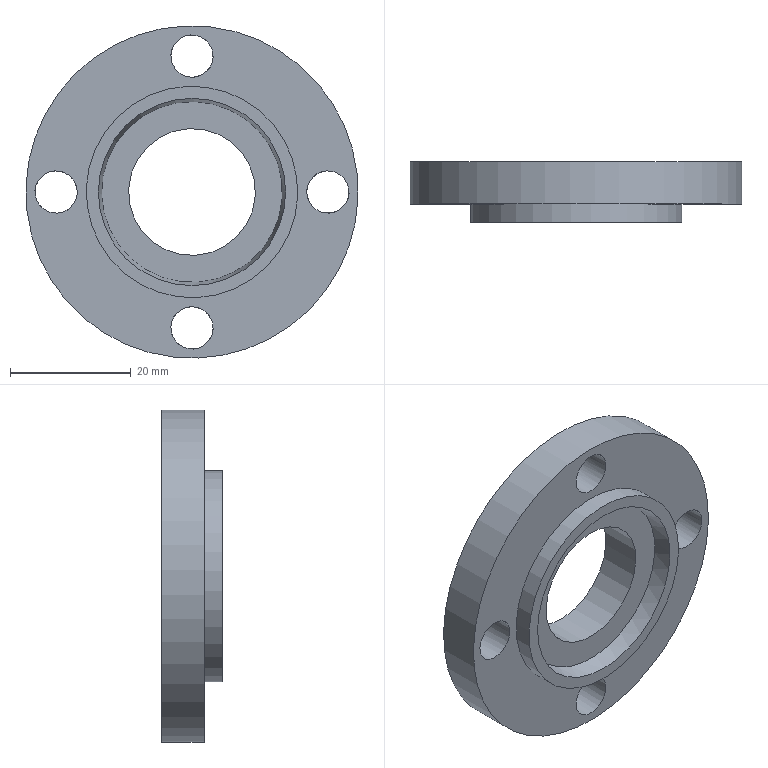Component | NX | BEARING_END_CAP_2 | 1 solid | 12 faces | box 55 x 10 x 55 mm | volume 13827 mm3 | cylinder 7 | plane 4 | cone 1 | commonest cylinder face diameters 7 x4 21 x1 35 x1 55 x1
STEP:
#1=CARTESIAN_POINT('',(0.,0.,0.));
#2=DIRECTION('',(0.,0.,1.));
#3=DIRECTION('',(1.,0.,0.));
#4=AXIS2_PLACEMENT_3D('',#1,#2,#3);
#5=CARTESIAN_POINT('',(626.689,-258.302,-1453.5));
#6=VERTEX_POINT('',#5);
#7=CARTESIAN_POINT('',(627.714,-258.302,-1451.025));
#8=VERTEX_POINT('',#7);
#9=CARTESIAN_POINT('',(630.189,-258.302,-1453.5));
#10=DIRECTION('',(0.,1.,0.));
#11=DIRECTION('',(-1.,0.,0.));
#12=AXIS2_PLACEMENT_3D('',#9,#10,#11);
#13=CIRCLE('',#12,3.5);
#14=CARTESIAN_POINT('',(610.744,-258.302,-1456.555));
#15=DIRECTION('',(0.,-1.,0.));
#16=DIRECTION('',(0.7071,0.,-0.7071));
#17=AXIS2_PLACEMENT_3D('',#14,#15,#16);
#18=PLANE('',#17);
#19=CARTESIAN_POINT('',(9.115,13.435));
#20=CARTESIAN_POINT('',(4.829,17.722));
#21=CARTESIAN_POINT('',(10.684,19.291));
#22=CARTESIAN_POINT('',(16.54,20.86));
#23=CARTESIAN_POINT('',(14.971,15.004));
#24=CARTESIAN_POINT('',(13.402,9.148));
#25=CARTESIAN_POINT('',(9.115,13.435));
#26=(BOUNDED_CURVE()B_SPLINE_CURVE(2,(#19,#20,#21,#22,#23,#24,#25),.UNSPECIFIED.,.T.,.F.)B_SPLINE_CURVE_WITH_KNOTS((1,2,2,2,2,1),(-2.094,0.,2.094,4.189,6.283,8.378),.UNSPECIFIED.)CURVE()GEOMETRIC_REPRESENTATION_ITEM()RATIONAL_B_SPLINE_CURVE((1.,0.5,1.,0.5,1.,0.5,1.))REPRESENTATION_ITEM(''));
#27=(GEOMETRIC_REPRESENTATION_CONTEXT(2)PARAMETRIC_REPRESENTATION_CONTEXT()REPRESENTATION_CONTEXT('',''));
#28=DEFINITIONAL_REPRESENTATION('',(#26),#27);
#29=PCURVE('',#18,#28);
#30=CARTESIAN_POINT('',(630.189,-281.302,-1453.5));
#31=DIRECTION('',(0.,1.,0.));
#32=DIRECTION('',(-0.7071,0.,0.7071));
#33=AXIS2_PLACEMENT_3D('',#30,#31,#32);
#34=CYLINDRICAL_SURFACE('',#33,3.5);
#35=CARTESIAN_POINT('',(5.498,23.));
#36=DIRECTION('',(1.,0.));
#37=VECTOR('',#36,1.);
#38=LINE('',#35,#37);
#39=(GEOMETRIC_REPRESENTATION_CONTEXT(2)PARAMETRIC_REPRESENTATION_CONTEXT()REPRESENTATION_CONTEXT('',''));
#40=DEFINITIONAL_REPRESENTATION('',(#38),#39);
#41=PCURVE('',#34,#40);
#42=SURFACE_CURVE('',#13,(#29,#41),.PCURVE_S1.);
#43=EDGE_CURVE('',#6,#8,#42,.T.);
#44=ORIENTED_EDGE('',*,*,#43,.F.);
#45=CARTESIAN_POINT('',(630.189,-258.302,-1453.5));
#46=DIRECTION('',(0.,1.,0.));
#47=DIRECTION('',(-1.,0.,0.));
#48=AXIS2_PLACEMENT_3D('',#45,#46,#47);
#49=CIRCLE('',#48,3.5);
#50=CARTESIAN_POINT('',(9.115,13.435));
#51=CARTESIAN_POINT('',(4.829,17.722));
#52=CARTESIAN_POINT('',(10.684,19.291));
#53=CARTESIAN_POINT('',(16.54,20.86));
#54=CARTESIAN_POINT('',(14.971,15.004));
#55=CARTESIAN_POINT('',(13.402,9.148));
#56=CARTESIAN_POINT('',(9.115,13.435));
#57=(BOUNDED_CURVE()B_SPLINE_CURVE(2,(#50,#51,#52,#53,#54,#55,#56),.UNSPECIFIED.,.T.,.F.)B_SPLINE_CURVE_WITH_KNOTS((1,2,2,2,2,1),(-2.094,0.,2.094,4.189,6.283,8.378),.UNSPECIFIED.)CURVE()GEOMETRIC_REPRESENTATION_ITEM()RATIONAL_B_SPLINE_CURVE((1.,0.5,1.,0.5,1.,0.5,1.))REPRESENTATION_ITEM(''));
#58=(GEOMETRIC_REPRESENTATION_CONTEXT(2)PARAMETRIC_REPRESENTATION_CONTEXT()REPRESENTATION_CONTEXT('',''));
#59=DEFINITIONAL_REPRESENTATION('',(#57),#58);
#60=PCURVE('',#18,#59);
#61=CARTESIAN_POINT('',(-0.7854,23.));
#62=DIRECTION('',(1.,0.));
#63=VECTOR('',#62,1.);
#64=LINE('',#61,#63);
#65=(GEOMETRIC_REPRESENTATION_CONTEXT(2)PARAMETRIC_REPRESENTATION_CONTEXT()REPRESENTATION_CONTEXT('',''));
#66=DEFINITIONAL_REPRESENTATION('',(#64),#65);
#67=PCURVE('',#34,#66);
#68=SURFACE_CURVE('',#49,(#60,#67),.PCURVE_S1.);
#69=EDGE_CURVE('',#8,#6,#68,.T.);
#70=ORIENTED_EDGE('',*,*,#69,.F.);
#71=EDGE_LOOP('',(#44,#70));
#72=FACE_BOUND('',#71,.T.);
#73=CARTESIAN_POINT('',(607.689,-258.302,-1479.5));
#74=VERTEX_POINT('',#73);
#75=CARTESIAN_POINT('',(605.214,-258.302,-1473.525));
#76=VERTEX_POINT('',#75);
#77=CARTESIAN_POINT('',(607.689,-258.302,-1476.));
#78=DIRECTION('',(0.,1.,0.));
#79=DIRECTION('',(0.,0.,-1.));
#80=AXIS2_PLACEMENT_3D('',#77,#78,#79);
#81=CIRCLE('',#80,3.5);
#82=CARTESIAN_POINT('',(14.065,-18.385));
#83=CARTESIAN_POINT('',(9.778,-22.671));
#84=CARTESIAN_POINT('',(8.209,-16.816));
#85=CARTESIAN_POINT('',(6.64,-10.96));
#86=CARTESIAN_POINT('',(12.496,-12.529));
#87=CARTESIAN_POINT('',(18.352,-14.098));
#88=CARTESIAN_POINT('',(14.065,-18.385));
#89=(BOUNDED_CURVE()B_SPLINE_CURVE(2,(#82,#83,#84,#85,#86,#87,#88),.UNSPECIFIED.,.T.,.F.)B_SPLINE_CURVE_WITH_KNOTS((1,2,2,2,2,1),(-2.094,0.,2.094,4.189,6.283,8.378),.UNSPECIFIED.)CURVE()GEOMETRIC_REPRESENTATION_ITEM()RATIONAL_B_SPLINE_CURVE((1.,0.5,1.,0.5,1.,0.5,1.))REPRESENTATION_ITEM(''));
#90=(GEOMETRIC_REPRESENTATION_CONTEXT(2)PARAMETRIC_REPRESENTATION_CONTEXT()REPRESENTATION_CONTEXT('',''));
#91=DEFINITIONAL_REPRESENTATION('',(#89),#90);
#92=PCURVE('',#18,#91);
#93=CARTESIAN_POINT('',(607.689,-281.302,-1476.));
#94=DIRECTION('',(0.,1.,0.));
#95=DIRECTION('',(-0.7071,0.,0.7071));
#96=AXIS2_PLACEMENT_3D('',#93,#94,#95);
#97=CYLINDRICAL_SURFACE('',#96,3.5);
#98=CARTESIAN_POINT('',(3.927,23.));
#99=DIRECTION('',(1.,0.));
#100=VECTOR('',#99,1.);
#101=LINE('',#98,#100);
#102=(GEOMETRIC_REPRESENTATION_CONTEXT(2)PARAMETRIC_REPRESENTATION_CONTEXT()REPRESENTATION_CONTEXT('',''));
#103=DEFINITIONAL_REPRESENTATION('',(#101),#102);
#104=PCURVE('',#97,#103);
#105=SURFACE_CURVE('',#81,(#92,#104),.PCURVE_S1.);
#106=EDGE_CURVE('',#74,#76,#105,.T.);
#107=ORIENTED_EDGE('',*,*,#106,.F.);
#108=CARTESIAN_POINT('',(607.689,-258.302,-1476.));
#109=DIRECTION('',(0.,1.,0.));
#110=DIRECTION('',(0.,0.,-1.));
#111=AXIS2_PLACEMENT_3D('',#108,#109,#110);
#112=CIRCLE('',#111,3.5);
#113=CARTESIAN_POINT('',(14.065,-18.385));
#114=CARTESIAN_POINT('',(9.778,-22.671));
#115=CARTESIAN_POINT('',(8.209,-16.816));
#116=CARTESIAN_POINT('',(6.64,-10.96));
#117=CARTESIAN_POINT('',(12.496,-12.529));
#118=CARTESIAN_POINT('',(18.352,-14.098));
#119=CARTESIAN_POINT('',(14.065,-18.385));
#120=(BOUNDED_CURVE()B_SPLINE_CURVE(2,(#113,#114,#115,#116,#117,#118,#119),.UNSPECIFIED.,.T.,.F.)B_SPLINE_CURVE_WITH_KNOTS((1,2,2,2,2,1),(-2.094,0.,2.094,4.189,6.283,8.378),.UNSPECIFIED.)CURVE()GEOMETRIC_REPRESENTATION_ITEM()RATIONAL_B_SPLINE_CURVE((1.,0.5,1.,0.5,1.,0.5,1.))REPRESENTATION_ITEM(''));
#121=(GEOMETRIC_REPRESENTATION_CONTEXT(2)PARAMETRIC_REPRESENTATION_CONTEXT()REPRESENTATION_CONTEXT('',''));
#122=DEFINITIONAL_REPRESENTATION('',(#120),#121);
#123=PCURVE('',#18,#122);
#124=CARTESIAN_POINT('',(-2.356,23.));
#125=DIRECTION('',(1.,0.));
#126=VECTOR('',#125,1.);
#127=LINE('',#124,#126);
#128=(GEOMETRIC_REPRESENTATION_CONTEXT(2)PARAMETRIC_REPRESENTATION_CONTEXT()REPRESENTATION_CONTEXT('',''));
#129=DEFINITIONAL_REPRESENTATION('',(#127),#128);
#130=PCURVE('',#97,#129);
#131=SURFACE_CURVE('',#112,(#123,#130),.PCURVE_S1.);
#132=EDGE_CURVE('',#76,#74,#131,.T.);
#133=ORIENTED_EDGE('',*,*,#132,.F.);
#134=EDGE_LOOP('',(#107,#133));
#135=FACE_BOUND('',#134,.T.);
#136=CARTESIAN_POINT('',(633.689,-258.302,-1498.5));
#137=VERTEX_POINT('',#136);
#138=CARTESIAN_POINT('',(627.714,-258.302,-1496.025));
#139=VERTEX_POINT('',#138);
#140=CARTESIAN_POINT('',(630.189,-258.302,-1498.5));
#141=DIRECTION('',(0.,1.,0.));
#142=DIRECTION('',(1.,0.,0.));
#143=AXIS2_PLACEMENT_3D('',#140,#141,#142);
#144=CIRCLE('',#143,3.5);
#145=CARTESIAN_POINT('',(45.885,-13.435));
#146=CARTESIAN_POINT('',(50.171,-17.722));
#147=CARTESIAN_POINT('',(44.316,-19.291));
#148=CARTESIAN_POINT('',(38.46,-20.86));
#149=CARTESIAN_POINT('',(40.029,-15.004));
#150=CARTESIAN_POINT('',(41.598,-9.148));
#151=CARTESIAN_POINT('',(45.885,-13.435));
#152=(BOUNDED_CURVE()B_SPLINE_CURVE(2,(#145,#146,#147,#148,#149,#150,#151),.UNSPECIFIED.,.T.,.F.)B_SPLINE_CURVE_WITH_KNOTS((1,2,2,2,2,1),(-2.094,0.,2.094,4.189,6.283,8.378),.UNSPECIFIED.)CURVE()GEOMETRIC_REPRESENTATION_ITEM()RATIONAL_B_SPLINE_CURVE((1.,0.5,1.,0.5,1.,0.5,1.))REPRESENTATION_ITEM(''));
#153=(GEOMETRIC_REPRESENTATION_CONTEXT(2)PARAMETRIC_REPRESENTATION_CONTEXT()REPRESENTATION_CONTEXT('',''));
#154=DEFINITIONAL_REPRESENTATION('',(#152),#153);
#155=PCURVE('',#18,#154);
#156=CARTESIAN_POINT('',(630.189,-281.302,-1498.5));
#157=DIRECTION('',(0.,1.,0.));
#158=DIRECTION('',(-0.7071,0.,0.7071));
#159=AXIS2_PLACEMENT_3D('',#156,#157,#158);
#160=CYLINDRICAL_SURFACE('',#159,3.5);
#161=CARTESIAN_POINT('',(2.356,23.));
#162=DIRECTION('',(1.,0.));
#163=VECTOR('',#162,1.);
#164=LINE('',#161,#163);
#165=(GEOMETRIC_REPRESENTATION_CONTEXT(2)PARAMETRIC_REPRESENTATION_CONTEXT()REPRESENTATION_CONTEXT('',''));
#166=DEFINITIONAL_REPRESENTATION('',(#164),#165);
#167=PCURVE('',#160,#166);
#168=SURFACE_CURVE('',#144,(#155,#167),.PCURVE_S1.);
#169=EDGE_CURVE('',#137,#139,#168,.T.);
#170=ORIENTED_EDGE('',*,*,#169,.F.);
#171=CARTESIAN_POINT('',(630.189,-258.302,-1498.5));
#172=DIRECTION('',(0.,1.,0.));
#173=DIRECTION('',(1.,0.,0.));
#174=AXIS2_PLACEMENT_3D('',#171,#172,#173);
#175=CIRCLE('',#174,3.5);
#176=CARTESIAN_POINT('',(45.885,-13.435));
#177=CARTESIAN_POINT('',(50.171,-17.722));
#178=CARTESIAN_POINT('',(44.316,-19.291));
#179=CARTESIAN_POINT('',(38.46,-20.86));
#180=CARTESIAN_POINT('',(40.029,-15.004));
#181=CARTESIAN_POINT('',(41.598,-9.148));
#182=CARTESIAN_POINT('',(45.885,-13.435));
#183=(BOUNDED_CURVE()B_SPLINE_CURVE(2,(#176,#177,#178,#179,#180,#181,#182),.UNSPECIFIED.,.T.,.F.)B_SPLINE_CURVE_WITH_KNOTS((1,2,2,2,2,1),(-2.094,0.,2.094,4.189,6.283,8.378),.UNSPECIFIED.)CURVE()GEOMETRIC_REPRESENTATION_ITEM()RATIONAL_B_SPLINE_CURVE((1.,0.5,1.,0.5,1.,0.5,1.))REPRESENTATION_ITEM(''));
#184=(GEOMETRIC_REPRESENTATION_CONTEXT(2)PARAMETRIC_REPRESENTATION_CONTEXT()REPRESENTATION_CONTEXT('',''));
#185=DEFINITIONAL_REPRESENTATION('',(#183),#184);
#186=PCURVE('',#18,#185);
#187=CARTESIAN_POINT('',(-3.927,23.));
#188=DIRECTION('',(1.,0.));
#189=VECTOR('',#188,1.);
#190=LINE('',#187,#189);
#191=(GEOMETRIC_REPRESENTATION_CONTEXT(2)PARAMETRIC_REPRESENTATION_CONTEXT()REPRESENTATION_CONTEXT('',''));
#192=DEFINITIONAL_REPRESENTATION('',(#190),#191);
#193=PCURVE('',#160,#192);
#194=SURFACE_CURVE('',#175,(#186,#193),.PCURVE_S1.);
#195=EDGE_CURVE('',#139,#137,#194,.T.);
#196=ORIENTED_EDGE('',*,*,#195,.F.);
#197=EDGE_LOOP('',(#170,#196));
#198=FACE_BOUND('',#197,.T.);
#199=CARTESIAN_POINT('',(652.689,-258.302,-1472.5));
#200=VERTEX_POINT('',#199);
#201=CARTESIAN_POINT('',(650.214,-258.302,-1473.525));
#202=VERTEX_POINT('',#201);
#203=CARTESIAN_POINT('',(652.689,-258.302,-1476.));
#204=DIRECTION('',(0.,1.,0.));
#205=DIRECTION('',(0.,0.,1.));
#206=AXIS2_PLACEMENT_3D('',#203,#204,#205);
#207=CIRCLE('',#206,3.5);
#208=CARTESIAN_POINT('',(40.935,18.385));
#209=CARTESIAN_POINT('',(45.222,22.671));
#210=CARTESIAN_POINT('',(46.791,16.816));
#211=CARTESIAN_POINT('',(48.36,10.96));
#212=CARTESIAN_POINT('',(42.504,12.529));
#213=CARTESIAN_POINT('',(36.648,14.098));
#214=CARTESIAN_POINT('',(40.935,18.385));
#215=(BOUNDED_CURVE()B_SPLINE_CURVE(2,(#208,#209,#210,#211,#212,#213,#214),.UNSPECIFIED.,.T.,.F.)B_SPLINE_CURVE_WITH_KNOTS((1,2,2,2,2,1),(-2.094,0.,2.094,4.189,6.283,8.378),.UNSPECIFIED.)CURVE()GEOMETRIC_REPRESENTATION_ITEM()RATIONAL_B_SPLINE_CURVE((1.,0.5,1.,0.5,1.,0.5,1.))REPRESENTATION_ITEM(''));
#216=(GEOMETRIC_REPRESENTATION_CONTEXT(2)PARAMETRIC_REPRESENTATION_CONTEXT()REPRESENTATION_CONTEXT('',''));
#217=DEFINITIONAL_REPRESENTATION('',(#215),#216);
#218=PCURVE('',#18,#217);
#219=CARTESIAN_POINT('',(652.689,-281.302,-1476.));
#220=DIRECTION('',(0.,1.,0.));
#221=DIRECTION('',(-0.7071,0.,0.7071));
#222=AXIS2_PLACEMENT_3D('',#219,#220,#221);
#223=CYLINDRICAL_SURFACE('',#222,3.5);
#224=CARTESIAN_POINT('',(0.7854,23.));
#225=DIRECTION('',(1.,0.));
#226=VECTOR('',#225,1.);
#227=LINE('',#224,#226);
#228=(GEOMETRIC_REPRESENTATION_CONTEXT(2)PARAMETRIC_REPRESENTATION_CONTEXT()REPRESENTATION_CONTEXT('',''));
#229=DEFINITIONAL_REPRESENTATION('',(#227),#228);
#230=PCURVE('',#223,#229);
#231=SURFACE_CURVE('',#207,(#218,#230),.PCURVE_S1.);
#232=EDGE_CURVE('',#200,#202,#231,.T.);
#233=ORIENTED_EDGE('',*,*,#232,.F.);
#234=CARTESIAN_POINT('',(652.689,-258.302,-1476.));
#235=DIRECTION('',(0.,1.,0.));
#236=DIRECTION('',(0.,0.,1.));
#237=AXIS2_PLACEMENT_3D('',#234,#235,#236);
#238=CIRCLE('',#237,3.5);
#239=CARTESIAN_POINT('',(40.935,18.385));
#240=CARTESIAN_POINT('',(45.222,22.671));
#241=CARTESIAN_POINT('',(46.791,16.816));
#242=CARTESIAN_POINT('',(48.36,10.96));
#243=CARTESIAN_POINT('',(42.504,12.529));
#244=CARTESIAN_POINT('',(36.648,14.098));
#245=CARTESIAN_POINT('',(40.935,18.385));
#246=(BOUNDED_CURVE()B_SPLINE_CURVE(2,(#239,#240,#241,#242,#243,#244,#245),.UNSPECIFIED.,.T.,.F.)B_SPLINE_CURVE_WITH_KNOTS((1,2,2,2,2,1),(-2.094,0.,2.094,4.189,6.283,8.378),.UNSPECIFIED.)CURVE()GEOMETRIC_REPRESENTATION_ITEM()RATIONAL_B_SPLINE_CURVE((1.,0.5,1.,0.5,1.,0.5,1.))REPRESENTATION_ITEM(''));
#247=(GEOMETRIC_REPRESENTATION_CONTEXT(2)PARAMETRIC_REPRESENTATION_CONTEXT()REPRESENTATION_CONTEXT('',''));
#248=DEFINITIONAL_REPRESENTATION('',(#246),#247);
#249=PCURVE('',#18,#248);
#250=CARTESIAN_POINT('',(-5.498,23.));
#251=DIRECTION('',(1.,0.));
#252=VECTOR('',#251,1.);
#253=LINE('',#250,#252);
#254=(GEOMETRIC_REPRESENTATION_CONTEXT(2)PARAMETRIC_REPRESENTATION_CONTEXT()REPRESENTATION_CONTEXT('',''));
#255=DEFINITIONAL_REPRESENTATION('',(#253),#254);
#256=PCURVE('',#223,#255);
#257=SURFACE_CURVE('',#238,(#249,#256),.PCURVE_S1.);
#258=EDGE_CURVE('',#202,#200,#257,.T.);
#259=ORIENTED_EDGE('',*,*,#258,.F.);
#260=EDGE_LOOP('',(#233,#259));
#261=FACE_BOUND('',#260,.T.);
#262=CARTESIAN_POINT('',(622.764,-258.302,-1468.575));
#263=VERTEX_POINT('',#262);
#264=CARTESIAN_POINT('',(630.189,-258.302,-1476.));
#265=DIRECTION('',(0.,1.,0.));
#266=DIRECTION('',(-0.7071,0.,0.7071));
#267=AXIS2_PLACEMENT_3D('',#264,#265,#266);
#268=CIRCLE('',#267,10.5);
#269=CARTESIAN_POINT('',(17.,0.));
#270=CARTESIAN_POINT('',(17.,18.187));
#271=CARTESIAN_POINT('',(32.75,9.093));
#272=CARTESIAN_POINT('',(48.5,0.));
#273=CARTESIAN_POINT('',(32.75,-9.093));
#274=CARTESIAN_POINT('',(17.,-18.187));
#275=CARTESIAN_POINT('',(17.,0.));
#276=(BOUNDED_CURVE()B_SPLINE_CURVE(2,(#269,#270,#271,#272,#273,#274,#275),.UNSPECIFIED.,.T.,.F.)B_SPLINE_CURVE_WITH_KNOTS((1,2,2,2,2,1),(-2.094,0.,2.094,4.189,6.283,8.378),.UNSPECIFIED.)CURVE()GEOMETRIC_REPRESENTATION_ITEM()RATIONAL_B_SPLINE_CURVE((1.,0.5,1.,0.5,1.,0.5,1.))REPRESENTATION_ITEM(''));
#277=(GEOMETRIC_REPRESENTATION_CONTEXT(2)PARAMETRIC_REPRESENTATION_CONTEXT()REPRESENTATION_CONTEXT('',''));
#278=DEFINITIONAL_REPRESENTATION('',(#276),#277);
#279=PCURVE('',#18,#278);
#280=CARTESIAN_POINT('',(630.189,-258.302,-1476.));
#281=DIRECTION('',(0.,1.,0.));
#282=DIRECTION('',(-0.7071,0.,0.7071));
#283=AXIS2_PLACEMENT_3D('',#280,#281,#282);
#284=CYLINDRICAL_SURFACE('',#283,10.5);
#285=CARTESIAN_POINT('',(0.,0.));
#286=DIRECTION('',(1.,0.));
#287=VECTOR('',#286,1.);
#288=LINE('',#285,#287);
#289=(GEOMETRIC_REPRESENTATION_CONTEXT(2)PARAMETRIC_REPRESENTATION_CONTEXT()REPRESENTATION_CONTEXT('',''));
#290=DEFINITIONAL_REPRESENTATION('',(#288),#289);
#291=PCURVE('',#284,#290);
#292=SURFACE_CURVE('',#268,(#279,#291),.PCURVE_S1.);
#293=EDGE_CURVE('',#263,#263,#292,.T.);
#294=ORIENTED_EDGE('',*,*,#293,.F.);
#295=EDGE_LOOP('',(#294));
#296=FACE_BOUND('',#295,.T.);
#297=CARTESIAN_POINT('',(610.744,-258.302,-1456.555));
#298=VERTEX_POINT('',#297);
#299=CARTESIAN_POINT('',(630.189,-258.302,-1476.));
#300=DIRECTION('',(0.,1.,0.));
#301=DIRECTION('',(-0.7071,0.,0.7071));
#302=AXIS2_PLACEMENT_3D('',#299,#300,#301);
#303=CIRCLE('',#302,27.5);
#304=CARTESIAN_POINT('',(-0.,0.));
#305=CARTESIAN_POINT('',(-0.,47.631));
#306=CARTESIAN_POINT('',(41.25,23.816));
#307=CARTESIAN_POINT('',(82.5,0.));
#308=CARTESIAN_POINT('',(41.25,-23.816));
#309=CARTESIAN_POINT('',(-0.,-47.631));
#310=CARTESIAN_POINT('',(-0.,0.));
#311=(BOUNDED_CURVE()B_SPLINE_CURVE(2,(#304,#305,#306,#307,#308,#309,#310),.UNSPECIFIED.,.T.,.F.)B_SPLINE_CURVE_WITH_KNOTS((1,2,2,2,2,1),(-2.094,0.,2.094,4.189,6.283,8.378),.UNSPECIFIED.)CURVE()GEOMETRIC_REPRESENTATION_ITEM()RATIONAL_B_SPLINE_CURVE((1.,0.5,1.,0.5,1.,0.5,1.))REPRESENTATION_ITEM(''));
#312=(GEOMETRIC_REPRESENTATION_CONTEXT(2)PARAMETRIC_REPRESENTATION_CONTEXT()REPRESENTATION_CONTEXT('',''));
#313=DEFINITIONAL_REPRESENTATION('',(#311),#312);
#314=PCURVE('',#18,#313);
#315=CARTESIAN_POINT('',(630.189,-258.302,-1476.));
#316=DIRECTION('',(0.,1.,0.));
#317=DIRECTION('',(-0.7071,0.,0.7071));
#318=AXIS2_PLACEMENT_3D('',#315,#316,#317);
#319=CYLINDRICAL_SURFACE('',#318,27.5);
#320=CARTESIAN_POINT('',(0.,0.));
#321=DIRECTION('',(1.,0.));
#322=VECTOR('',#321,1.);
#323=LINE('',#320,#322);
#324=(GEOMETRIC_REPRESENTATION_CONTEXT(2)PARAMETRIC_REPRESENTATION_CONTEXT()REPRESENTATION_CONTEXT('',''));
#325=DEFINITIONAL_REPRESENTATION('',(#323),#324);
#326=PCURVE('',#319,#325);
#327=SURFACE_CURVE('',#303,(#314,#326),.PCURVE_S1.);
#328=EDGE_CURVE('',#298,#298,#327,.T.);
#329=ORIENTED_EDGE('',*,*,#328,.T.);
#330=EDGE_LOOP('',(#329));
#331=FACE_BOUND('',#330,.T.);
#332=ADVANCED_FACE('',(#72,#135,#198,#261,#296,#331),#18,.F.);
#333=CARTESIAN_POINT('',(622.764,-265.302,-1468.575));
#334=VERTEX_POINT('',#333);
#335=CARTESIAN_POINT('',(630.189,-265.302,-1476.));
#336=DIRECTION('',(0.,1.,0.));
#337=DIRECTION('',(-0.7071,0.,0.7071));
#338=AXIS2_PLACEMENT_3D('',#335,#336,#337);
#339=CIRCLE('',#338,10.5);
#340=CARTESIAN_POINT('',(0.,-7.));
#341=DIRECTION('',(1.,0.));
#342=VECTOR('',#341,1.);
#343=LINE('',#340,#342);
#344=(GEOMETRIC_REPRESENTATION_CONTEXT(2)PARAMETRIC_REPRESENTATION_CONTEXT()REPRESENTATION_CONTEXT('',''));
#345=DEFINITIONAL_REPRESENTATION('',(#343),#344);
#346=PCURVE('',#284,#345);
#347=CARTESIAN_POINT('',(622.764,-265.302,-1468.575));
#348=DIRECTION('',(0.,1.,0.));
#349=DIRECTION('',(-0.7071,0.,0.7071));
#350=AXIS2_PLACEMENT_3D('',#347,#348,#349);
#351=PLANE('',#350);
#352=CARTESIAN_POINT('',(-10.5,-0.));
#353=DIRECTION('',(1.,-0.));
#354=AXIS2_PLACEMENT_2D('',#352,#353);
#355=CIRCLE('',#354,10.5);
#356=(GEOMETRIC_REPRESENTATION_CONTEXT(2)PARAMETRIC_REPRESENTATION_CONTEXT()REPRESENTATION_CONTEXT('',''));
#357=DEFINITIONAL_REPRESENTATION('',(#355),#356);
#358=PCURVE('',#351,#357);
#359=SURFACE_CURVE('',#339,(#346,#358),.PCURVE_S1.);
#360=EDGE_CURVE('',#334,#334,#359,.T.);
#361=ORIENTED_EDGE('',*,*,#360,.T.);
#362=CARTESIAN_POINT('',(622.764,-265.302,-1468.575));
#363=CARTESIAN_POINT('',(622.764,-258.302,-1468.575));
#364=B_SPLINE_CURVE_WITH_KNOTS('',1,(#362,#363),.UNSPECIFIED.,.F.,.F.,(2,2),(-7.,0.),.PIECEWISE_BEZIER_KNOTS.);
#365=CARTESIAN_POINT('',(6.283,0.));
#366=DIRECTION('',(0.,1.));
#367=VECTOR('',#366,1.);
#368=LINE('',#365,#367);
#369=(GEOMETRIC_REPRESENTATION_CONTEXT(2)PARAMETRIC_REPRESENTATION_CONTEXT()REPRESENTATION_CONTEXT('',''));
#370=DEFINITIONAL_REPRESENTATION('',(#368),#369);
#371=PCURVE('',#284,#370);
#372=CARTESIAN_POINT('',(0.,0.));
#373=DIRECTION('',(0.,1.));
#374=VECTOR('',#373,1.);
#375=LINE('',#372,#374);
#376=(GEOMETRIC_REPRESENTATION_CONTEXT(2)PARAMETRIC_REPRESENTATION_CONTEXT()REPRESENTATION_CONTEXT('',''));
#377=DEFINITIONAL_REPRESENTATION('',(#375),#376);
#378=PCURVE('',#284,#377);
#379=SEAM_CURVE('',#364,(#371,#378),.PCURVE_S1.);
#380=EDGE_CURVE('',#334,#263,#379,.T.);
#381=ORIENTED_EDGE('',*,*,#380,.T.);
#382=ORIENTED_EDGE('',*,*,#293,.F.);
#383=ORIENTED_EDGE('',*,*,#380,.F.);
#384=EDGE_LOOP('',(#361,#381,#382,#383));
#385=FACE_BOUND('',#384,.F.);
#386=ADVANCED_FACE('',(#385),#284,.F.);
#387=CARTESIAN_POINT('',(619.603,-265.302,-1465.414));
#388=VERTEX_POINT('',#387);
#389=CARTESIAN_POINT('',(630.189,-265.302,-1476.));
#390=DIRECTION('',(0.,1.,0.));
#391=DIRECTION('',(-0.7071,0.,0.7071));
#392=AXIS2_PLACEMENT_3D('',#389,#390,#391);
#393=CIRCLE('',#392,14.971);
#394=CARTESIAN_POINT('',(-10.5,-0.));
#395=DIRECTION('',(1.,0.));
#396=AXIS2_PLACEMENT_2D('',#394,#395);
#397=CIRCLE('',#396,14.971);
#398=(GEOMETRIC_REPRESENTATION_CONTEXT(2)PARAMETRIC_REPRESENTATION_CONTEXT()REPRESENTATION_CONTEXT('',''));
#399=DEFINITIONAL_REPRESENTATION('',(#397),#398);
#400=PCURVE('',#351,#399);
#401=CARTESIAN_POINT('',(630.189,-265.302,-1476.));
#402=DIRECTION('',(0.,-1.,0.));
#403=DIRECTION('',(0.7071,0.,-0.7071));
#404=AXIS2_PLACEMENT_3D('',#401,#402,#403);
#405=CONICAL_SURFACE('',#404,14.971,0.1745);
#406=CARTESIAN_POINT('',(9.425,-0.));
#407=DIRECTION('',(-1.,0.));
#408=VECTOR('',#407,1.);
#409=LINE('',#406,#408);
#410=(GEOMETRIC_REPRESENTATION_CONTEXT(2)PARAMETRIC_REPRESENTATION_CONTEXT()REPRESENTATION_CONTEXT('',''));
#411=DEFINITIONAL_REPRESENTATION('',(#409),#410);
#412=PCURVE('',#405,#411);
#413=SURFACE_CURVE('',#393,(#400,#412),.PCURVE_S1.);
#414=EDGE_CURVE('',#388,#388,#413,.T.);
#415=ORIENTED_EDGE('',*,*,#414,.F.);
#416=EDGE_LOOP('',(#415));
#417=FACE_BOUND('',#416,.T.);
#418=ORIENTED_EDGE('',*,*,#360,.T.);
#419=EDGE_LOOP('',(#418));
#420=FACE_BOUND('',#419,.T.);
#421=ADVANCED_FACE('',(#417,#420),#351,.F.);
#422=CARTESIAN_POINT('',(619.229,-268.302,-1465.04));
#423=VERTEX_POINT('',#422);
#424=CARTESIAN_POINT('',(630.189,-268.302,-1476.));
#425=DIRECTION('',(0.,1.,0.));
#426=DIRECTION('',(-0.7071,0.,0.7071));
#427=AXIS2_PLACEMENT_3D('',#424,#425,#426);
#428=CIRCLE('',#427,15.5);
#429=CARTESIAN_POINT('',(9.425,3.));
#430=DIRECTION('',(-1.,0.));
#431=VECTOR('',#430,1.);
#432=LINE('',#429,#431);
#433=(GEOMETRIC_REPRESENTATION_CONTEXT(2)PARAMETRIC_REPRESENTATION_CONTEXT()REPRESENTATION_CONTEXT('',''));
#434=DEFINITIONAL_REPRESENTATION('',(#432),#433);
#435=PCURVE('',#405,#434);
#436=CARTESIAN_POINT('',(619.229,-268.302,-1465.04));
#437=DIRECTION('',(0.,1.,0.));
#438=DIRECTION('',(-0.7071,0.,0.7071));
#439=AXIS2_PLACEMENT_3D('',#436,#437,#438);
#440=PLANE('',#439);
#441=CARTESIAN_POINT('',(-15.5,0.));
#442=DIRECTION('',(1.,0.));
#443=AXIS2_PLACEMENT_2D('',#441,#442);
#444=CIRCLE('',#443,15.5);
#445=(GEOMETRIC_REPRESENTATION_CONTEXT(2)PARAMETRIC_REPRESENTATION_CONTEXT()REPRESENTATION_CONTEXT('',''));
#446=DEFINITIONAL_REPRESENTATION('',(#444),#445);
#447=PCURVE('',#440,#446);
#448=SURFACE_CURVE('',#428,(#435,#447),.PCURVE_S1.);
#449=EDGE_CURVE('',#423,#423,#448,.T.);
#450=ORIENTED_EDGE('',*,*,#449,.T.);
#451=CARTESIAN_POINT('',(619.603,-265.302,-1465.414));
#452=CARTESIAN_POINT('',(619.229,-268.302,-1465.04));
#453=B_SPLINE_CURVE_WITH_KNOTS('',1,(#451,#452),.UNSPECIFIED.,.F.,.F.,(2,2),(-0.,3.046),.PIECEWISE_BEZIER_KNOTS.);
#454=CARTESIAN_POINT('',(3.142,0.));
#455=DIRECTION('',(0.,1.));
#456=VECTOR('',#455,1.);
#457=LINE('',#454,#456);
#458=(GEOMETRIC_REPRESENTATION_CONTEXT(2)PARAMETRIC_REPRESENTATION_CONTEXT()REPRESENTATION_CONTEXT('',''));
#459=DEFINITIONAL_REPRESENTATION('',(#457),#458);
#460=PCURVE('',#405,#459);
#461=CARTESIAN_POINT('',(9.425,0.));
#462=DIRECTION('',(0.,1.));
#463=VECTOR('',#462,1.);
#464=LINE('',#461,#463);
#465=(GEOMETRIC_REPRESENTATION_CONTEXT(2)PARAMETRIC_REPRESENTATION_CONTEXT()REPRESENTATION_CONTEXT('',''));
#466=DEFINITIONAL_REPRESENTATION('',(#464),#465);
#467=PCURVE('',#405,#466);
#468=SEAM_CURVE('',#453,(#460,#467),.PCURVE_S1.);
#469=EDGE_CURVE('',#388,#423,#468,.T.);
#470=ORIENTED_EDGE('',*,*,#469,.F.);
#471=ORIENTED_EDGE('',*,*,#414,.F.);
#472=ORIENTED_EDGE('',*,*,#469,.T.);
#473=EDGE_LOOP('',(#450,#470,#471,#472));
#474=FACE_BOUND('',#473,.F.);
#475=ADVANCED_FACE('',(#474),#405,.F.);
#476=CARTESIAN_POINT('',(617.815,-268.302,-1463.626));
#477=VERTEX_POINT('',#476);
#478=CARTESIAN_POINT('',(630.189,-268.302,-1476.));
#479=DIRECTION('',(0.,1.,0.));
#480=DIRECTION('',(-0.7071,0.,0.7071));
#481=AXIS2_PLACEMENT_3D('',#478,#479,#480);
#482=CIRCLE('',#481,17.5);
#483=CARTESIAN_POINT('',(-15.5,0.));
#484=DIRECTION('',(1.,0.));
#485=AXIS2_PLACEMENT_2D('',#483,#484);
#486=CIRCLE('',#485,17.5);
#487=(GEOMETRIC_REPRESENTATION_CONTEXT(2)PARAMETRIC_REPRESENTATION_CONTEXT()REPRESENTATION_CONTEXT('',''));
#488=DEFINITIONAL_REPRESENTATION('',(#486),#487);
#489=PCURVE('',#440,#488);
#490=CARTESIAN_POINT('',(630.189,-258.302,-1476.));
#491=DIRECTION('',(0.,1.,0.));
#492=DIRECTION('',(-0.7071,0.,0.7071));
#493=AXIS2_PLACEMENT_3D('',#490,#491,#492);
#494=CYLINDRICAL_SURFACE('',#493,17.5);
#495=CARTESIAN_POINT('',(0.,-10.));
#496=DIRECTION('',(1.,0.));
#497=VECTOR('',#496,1.);
#498=LINE('',#495,#497);
#499=(GEOMETRIC_REPRESENTATION_CONTEXT(2)PARAMETRIC_REPRESENTATION_CONTEXT()REPRESENTATION_CONTEXT('',''));
#500=DEFINITIONAL_REPRESENTATION('',(#498),#499);
#501=PCURVE('',#494,#500);
#502=SURFACE_CURVE('',#482,(#489,#501),.PCURVE_S1.);
#503=EDGE_CURVE('',#477,#477,#502,.T.);
#504=ORIENTED_EDGE('',*,*,#503,.F.);
#505=EDGE_LOOP('',(#504));
#506=FACE_BOUND('',#505,.T.);
#507=ORIENTED_EDGE('',*,*,#449,.T.);
#508=EDGE_LOOP('',(#507));
#509=FACE_BOUND('',#508,.T.);
#510=ADVANCED_FACE('',(#506,#509),#440,.F.);
#511=CARTESIAN_POINT('',(617.815,-265.302,-1463.626));
#512=VERTEX_POINT('',#511);
#513=CARTESIAN_POINT('',(630.189,-265.302,-1476.));
#514=DIRECTION('',(0.,1.,0.));
#515=DIRECTION('',(-0.7071,0.,0.7071));
#516=AXIS2_PLACEMENT_3D('',#513,#514,#515);
#517=CIRCLE('',#516,17.5);
#518=CARTESIAN_POINT('',(0.,-7.));
#519=DIRECTION('',(1.,0.));
#520=VECTOR('',#519,1.);
#521=LINE('',#518,#520);
#522=(GEOMETRIC_REPRESENTATION_CONTEXT(2)PARAMETRIC_REPRESENTATION_CONTEXT()REPRESENTATION_CONTEXT('',''));
#523=DEFINITIONAL_REPRESENTATION('',(#521),#522);
#524=PCURVE('',#494,#523);
#525=CARTESIAN_POINT('',(617.815,-265.302,-1463.626));
#526=DIRECTION('',(0.,1.,0.));
#527=DIRECTION('',(-0.7071,0.,0.7071));
#528=AXIS2_PLACEMENT_3D('',#525,#526,#527);
#529=PLANE('',#528);
#530=CARTESIAN_POINT('',(-17.5,0.));
#531=DIRECTION('',(1.,0.));
#532=AXIS2_PLACEMENT_2D('',#530,#531);
#533=CIRCLE('',#532,17.5);
#534=(GEOMETRIC_REPRESENTATION_CONTEXT(2)PARAMETRIC_REPRESENTATION_CONTEXT()REPRESENTATION_CONTEXT('',''));
#535=DEFINITIONAL_REPRESENTATION('',(#533),#534);
#536=PCURVE('',#529,#535);
#537=SURFACE_CURVE('',#517,(#524,#536),.PCURVE_S1.);
#538=EDGE_CURVE('',#512,#512,#537,.T.);
#539=ORIENTED_EDGE('',*,*,#538,.F.);
#540=CARTESIAN_POINT('',(617.815,-268.302,-1463.626));
#541=CARTESIAN_POINT('',(617.815,-265.302,-1463.626));
#542=B_SPLINE_CURVE_WITH_KNOTS('',1,(#540,#541),.UNSPECIFIED.,.F.,.F.,(2,2),(-10.,-7.),.PIECEWISE_BEZIER_KNOTS.);
#543=CARTESIAN_POINT('',(0.,0.));
#544=DIRECTION('',(0.,1.));
#545=VECTOR('',#544,1.);
#546=LINE('',#543,#545);
#547=(GEOMETRIC_REPRESENTATION_CONTEXT(2)PARAMETRIC_REPRESENTATION_CONTEXT()REPRESENTATION_CONTEXT('',''));
#548=DEFINITIONAL_REPRESENTATION('',(#546),#547);
#549=PCURVE('',#494,#548);
#550=CARTESIAN_POINT('',(6.283,0.));
#551=DIRECTION('',(0.,1.));
#552=VECTOR('',#551,1.);
#553=LINE('',#550,#552);
#554=(GEOMETRIC_REPRESENTATION_CONTEXT(2)PARAMETRIC_REPRESENTATION_CONTEXT()REPRESENTATION_CONTEXT('',''));
#555=DEFINITIONAL_REPRESENTATION('',(#553),#554);
#556=PCURVE('',#494,#555);
#557=SEAM_CURVE('',#542,(#549,#556),.PCURVE_S1.);
#558=EDGE_CURVE('',#477,#512,#557,.T.);
#559=ORIENTED_EDGE('',*,*,#558,.F.);
#560=ORIENTED_EDGE('',*,*,#503,.T.);
#561=ORIENTED_EDGE('',*,*,#558,.T.);
#562=EDGE_LOOP('',(#539,#559,#560,#561));
#563=FACE_BOUND('',#562,.T.);
#564=ADVANCED_FACE('',(#563),#494,.T.);
#565=CARTESIAN_POINT('',(627.714,-265.302,-1451.025));
#566=VERTEX_POINT('',#565);
#567=CARTESIAN_POINT('',(630.189,-265.302,-1453.5));
#568=DIRECTION('',(0.,1.,0.));
#569=DIRECTION('',(-0.7071,0.,0.7071));
#570=AXIS2_PLACEMENT_3D('',#567,#568,#569);
#571=CIRCLE('',#570,3.5);
#572=CARTESIAN_POINT('',(-1.59,15.91));
#573=DIRECTION('',(1.,-0.));
#574=AXIS2_PLACEMENT_2D('',#572,#573);
#575=CIRCLE('',#574,3.5);
#576=(GEOMETRIC_REPRESENTATION_CONTEXT(2)PARAMETRIC_REPRESENTATION_CONTEXT()REPRESENTATION_CONTEXT('',''));
#577=DEFINITIONAL_REPRESENTATION('',(#575),#576);
#578=PCURVE('',#529,#577);
#579=CARTESIAN_POINT('',(0.,16.));
#580=DIRECTION('',(1.,0.));
#581=VECTOR('',#580,1.);
#582=LINE('',#579,#581);
#583=(GEOMETRIC_REPRESENTATION_CONTEXT(2)PARAMETRIC_REPRESENTATION_CONTEXT()REPRESENTATION_CONTEXT('',''));
#584=DEFINITIONAL_REPRESENTATION('',(#582),#583);
#585=PCURVE('',#34,#584);
#586=SURFACE_CURVE('',#571,(#578,#585),.PCURVE_S1.);
#587=EDGE_CURVE('',#566,#566,#586,.T.);
#588=ORIENTED_EDGE('',*,*,#587,.T.);
#589=EDGE_LOOP('',(#588));
#590=FACE_BOUND('',#589,.T.);
#591=CARTESIAN_POINT('',(605.214,-265.302,-1473.525));
#592=VERTEX_POINT('',#591);
#593=CARTESIAN_POINT('',(607.689,-265.302,-1476.));
#594=DIRECTION('',(0.,1.,0.));
#595=DIRECTION('',(-0.7071,0.,0.7071));
#596=AXIS2_PLACEMENT_3D('',#593,#594,#595);
#597=CIRCLE('',#596,3.5);
#598=CARTESIAN_POINT('',(-1.59,-15.91));
#599=DIRECTION('',(1.,-0.));
#600=AXIS2_PLACEMENT_2D('',#598,#599);
#601=CIRCLE('',#600,3.5);
#602=(GEOMETRIC_REPRESENTATION_CONTEXT(2)PARAMETRIC_REPRESENTATION_CONTEXT()REPRESENTATION_CONTEXT('',''));
#603=DEFINITIONAL_REPRESENTATION('',(#601),#602);
#604=PCURVE('',#529,#603);
#605=CARTESIAN_POINT('',(0.,16.));
#606=DIRECTION('',(1.,0.));
#607=VECTOR('',#606,1.);
#608=LINE('',#605,#607);
#609=(GEOMETRIC_REPRESENTATION_CONTEXT(2)PARAMETRIC_REPRESENTATION_CONTEXT()REPRESENTATION_CONTEXT('',''));
#610=DEFINITIONAL_REPRESENTATION('',(#608),#609);
#611=PCURVE('',#97,#610);
#612=SURFACE_CURVE('',#597,(#604,#611),.PCURVE_S1.);
#613=EDGE_CURVE('',#592,#592,#612,.T.);
#614=ORIENTED_EDGE('',*,*,#613,.T.);
#615=EDGE_LOOP('',(#614));
#616=FACE_BOUND('',#615,.T.);
#617=CARTESIAN_POINT('',(627.714,-265.302,-1496.025));
#618=VERTEX_POINT('',#617);
#619=CARTESIAN_POINT('',(630.189,-265.302,-1498.5));
#620=DIRECTION('',(0.,1.,0.));
#621=DIRECTION('',(-0.7071,0.,0.7071));
#622=AXIS2_PLACEMENT_3D('',#619,#620,#621);
#623=CIRCLE('',#622,3.5);
#624=CARTESIAN_POINT('',(-33.41,-15.91));
#625=DIRECTION('',(1.,-0.));
#626=AXIS2_PLACEMENT_2D('',#624,#625);
#627=CIRCLE('',#626,3.5);
#628=(GEOMETRIC_REPRESENTATION_CONTEXT(2)PARAMETRIC_REPRESENTATION_CONTEXT()REPRESENTATION_CONTEXT('',''));
#629=DEFINITIONAL_REPRESENTATION('',(#627),#628);
#630=PCURVE('',#529,#629);
#631=CARTESIAN_POINT('',(0.,16.));
#632=DIRECTION('',(1.,0.));
#633=VECTOR('',#632,1.);
#634=LINE('',#631,#633);
#635=(GEOMETRIC_REPRESENTATION_CONTEXT(2)PARAMETRIC_REPRESENTATION_CONTEXT()REPRESENTATION_CONTEXT('',''));
#636=DEFINITIONAL_REPRESENTATION('',(#634),#635);
#637=PCURVE('',#160,#636);
#638=SURFACE_CURVE('',#623,(#630,#637),.PCURVE_S1.);
#639=EDGE_CURVE('',#618,#618,#638,.T.);
#640=ORIENTED_EDGE('',*,*,#639,.T.);
#641=EDGE_LOOP('',(#640));
#642=FACE_BOUND('',#641,.T.);
#643=CARTESIAN_POINT('',(650.214,-265.302,-1473.525));
#644=VERTEX_POINT('',#643);
#645=CARTESIAN_POINT('',(652.689,-265.302,-1476.));
#646=DIRECTION('',(0.,1.,0.));
#647=DIRECTION('',(-0.7071,0.,0.7071));
#648=AXIS2_PLACEMENT_3D('',#645,#646,#647);
#649=CIRCLE('',#648,3.5);
#650=CARTESIAN_POINT('',(-33.41,15.91));
#651=DIRECTION('',(1.,-0.));
#652=AXIS2_PLACEMENT_2D('',#650,#651);
#653=CIRCLE('',#652,3.5);
#654=(GEOMETRIC_REPRESENTATION_CONTEXT(2)PARAMETRIC_REPRESENTATION_CONTEXT()REPRESENTATION_CONTEXT('',''));
#655=DEFINITIONAL_REPRESENTATION('',(#653),#654);
#656=PCURVE('',#529,#655);
#657=CARTESIAN_POINT('',(0.,16.));
#658=DIRECTION('',(1.,0.));
#659=VECTOR('',#658,1.);
#660=LINE('',#657,#659);
#661=(GEOMETRIC_REPRESENTATION_CONTEXT(2)PARAMETRIC_REPRESENTATION_CONTEXT()REPRESENTATION_CONTEXT('',''));
#662=DEFINITIONAL_REPRESENTATION('',(#660),#661);
#663=PCURVE('',#223,#662);
#664=SURFACE_CURVE('',#649,(#656,#663),.PCURVE_S1.);
#665=EDGE_CURVE('',#644,#644,#664,.T.);
#666=ORIENTED_EDGE('',*,*,#665,.T.);
#667=EDGE_LOOP('',(#666));
#668=FACE_BOUND('',#667,.T.);
#669=CARTESIAN_POINT('',(610.744,-265.302,-1456.555));
#670=VERTEX_POINT('',#669);
#671=CARTESIAN_POINT('',(630.189,-265.302,-1476.));
#672=DIRECTION('',(0.,1.,0.));
#673=DIRECTION('',(-0.7071,0.,0.7071));
#674=AXIS2_PLACEMENT_3D('',#671,#672,#673);
#675=CIRCLE('',#674,27.5);
#676=CARTESIAN_POINT('',(-17.5,0.));
#677=DIRECTION('',(1.,0.));
#678=AXIS2_PLACEMENT_2D('',#676,#677);
#679=CIRCLE('',#678,27.5);
#680=(GEOMETRIC_REPRESENTATION_CONTEXT(2)PARAMETRIC_REPRESENTATION_CONTEXT()REPRESENTATION_CONTEXT('',''));
#681=DEFINITIONAL_REPRESENTATION('',(#679),#680);
#682=PCURVE('',#529,#681);
#683=CARTESIAN_POINT('',(0.,-7.));
#684=DIRECTION('',(1.,0.));
#685=VECTOR('',#684,1.);
#686=LINE('',#683,#685);
#687=(GEOMETRIC_REPRESENTATION_CONTEXT(2)PARAMETRIC_REPRESENTATION_CONTEXT()REPRESENTATION_CONTEXT('',''));
#688=DEFINITIONAL_REPRESENTATION('',(#686),#687);
#689=PCURVE('',#319,#688);
#690=SURFACE_CURVE('',#675,(#682,#689),.PCURVE_S1.);
#691=EDGE_CURVE('',#670,#670,#690,.T.);
#692=ORIENTED_EDGE('',*,*,#691,.F.);
#693=EDGE_LOOP('',(#692));
#694=FACE_BOUND('',#693,.T.);
#695=ORIENTED_EDGE('',*,*,#538,.T.);
#696=EDGE_LOOP('',(#695));
#697=FACE_BOUND('',#696,.T.);
#698=ADVANCED_FACE('',(#590,#616,#642,#668,#694,#697),#529,.F.);
#699=ORIENTED_EDGE('',*,*,#328,.F.);
#700=CARTESIAN_POINT('',(610.744,-265.302,-1456.555));
#701=CARTESIAN_POINT('',(610.744,-258.302,-1456.555));
#702=B_SPLINE_CURVE_WITH_KNOTS('',1,(#700,#701),.UNSPECIFIED.,.F.,.F.,(2,2),(-7.,0.),.PIECEWISE_BEZIER_KNOTS.);
#703=CARTESIAN_POINT('',(0.,0.));
#704=DIRECTION('',(0.,1.));
#705=VECTOR('',#704,1.);
#706=LINE('',#703,#705);
#707=(GEOMETRIC_REPRESENTATION_CONTEXT(2)PARAMETRIC_REPRESENTATION_CONTEXT()REPRESENTATION_CONTEXT('',''));
#708=DEFINITIONAL_REPRESENTATION('',(#706),#707);
#709=PCURVE('',#319,#708);
#710=CARTESIAN_POINT('',(6.283,0.));
#711=DIRECTION('',(0.,1.));
#712=VECTOR('',#711,1.);
#713=LINE('',#710,#712);
#714=(GEOMETRIC_REPRESENTATION_CONTEXT(2)PARAMETRIC_REPRESENTATION_CONTEXT()REPRESENTATION_CONTEXT('',''));
#715=DEFINITIONAL_REPRESENTATION('',(#713),#714);
#716=PCURVE('',#319,#715);
#717=SEAM_CURVE('',#702,(#709,#716),.PCURVE_S1.);
#718=EDGE_CURVE('',#670,#298,#717,.T.);
#719=ORIENTED_EDGE('',*,*,#718,.F.);
#720=ORIENTED_EDGE('',*,*,#691,.T.);
#721=ORIENTED_EDGE('',*,*,#718,.T.);
#722=EDGE_LOOP('',(#699,#719,#720,#721));
#723=FACE_BOUND('',#722,.T.);
#724=ADVANCED_FACE('',(#723),#319,.T.);
#725=ORIENTED_EDGE('',*,*,#258,.F.);
#726=CARTESIAN_POINT('',(650.214,-265.302,-1473.525));
#727=CARTESIAN_POINT('',(650.214,-258.302,-1473.525));
#728=B_SPLINE_CURVE_WITH_KNOTS('',1,(#726,#727),.UNSPECIFIED.,.F.,.F.,(2,2),(16.,23.),.PIECEWISE_BEZIER_KNOTS.);
#729=CARTESIAN_POINT('',(0.,0.));
#730=DIRECTION('',(0.,1.));
#731=VECTOR('',#730,1.);
#732=LINE('',#729,#731);
#733=(GEOMETRIC_REPRESENTATION_CONTEXT(2)PARAMETRIC_REPRESENTATION_CONTEXT()REPRESENTATION_CONTEXT('',''));
#734=DEFINITIONAL_REPRESENTATION('',(#732),#733);
#735=PCURVE('',#223,#734);
#736=CARTESIAN_POINT('',(6.283,0.));
#737=DIRECTION('',(0.,1.));
#738=VECTOR('',#737,1.);
#739=LINE('',#736,#738);
#740=(GEOMETRIC_REPRESENTATION_CONTEXT(2)PARAMETRIC_REPRESENTATION_CONTEXT()REPRESENTATION_CONTEXT('',''));
#741=DEFINITIONAL_REPRESENTATION('',(#739),#740);
#742=PCURVE('',#223,#741);
#743=SEAM_CURVE('',#728,(#735,#742),.PCURVE_S1.);
#744=EDGE_CURVE('',#644,#202,#743,.T.);
#745=ORIENTED_EDGE('',*,*,#744,.F.);
#746=ORIENTED_EDGE('',*,*,#665,.T.);
#747=ORIENTED_EDGE('',*,*,#744,.T.);
#748=ORIENTED_EDGE('',*,*,#232,.F.);
#749=EDGE_LOOP('',(#725,#745,#746,#747,#748));
#750=FACE_BOUND('',#749,.F.);
#751=ADVANCED_FACE('',(#750),#223,.F.);
#752=ORIENTED_EDGE('',*,*,#195,.F.);
#753=CARTESIAN_POINT('',(627.714,-265.302,-1496.025));
#754=CARTESIAN_POINT('',(627.714,-258.302,-1496.025));
#755=B_SPLINE_CURVE_WITH_KNOTS('',1,(#753,#754),.UNSPECIFIED.,.F.,.F.,(2,2),(16.,23.),.PIECEWISE_BEZIER_KNOTS.);
#756=CARTESIAN_POINT('',(0.,0.));
#757=DIRECTION('',(0.,1.));
#758=VECTOR('',#757,1.);
#759=LINE('',#756,#758);
#760=(GEOMETRIC_REPRESENTATION_CONTEXT(2)PARAMETRIC_REPRESENTATION_CONTEXT()REPRESENTATION_CONTEXT('',''));
#761=DEFINITIONAL_REPRESENTATION('',(#759),#760);
#762=PCURVE('',#160,#761);
#763=CARTESIAN_POINT('',(6.283,0.));
#764=DIRECTION('',(0.,1.));
#765=VECTOR('',#764,1.);
#766=LINE('',#763,#765);
#767=(GEOMETRIC_REPRESENTATION_CONTEXT(2)PARAMETRIC_REPRESENTATION_CONTEXT()REPRESENTATION_CONTEXT('',''));
#768=DEFINITIONAL_REPRESENTATION('',(#766),#767);
#769=PCURVE('',#160,#768);
#770=SEAM_CURVE('',#755,(#762,#769),.PCURVE_S1.);
#771=EDGE_CURVE('',#618,#139,#770,.T.);
#772=ORIENTED_EDGE('',*,*,#771,.F.);
#773=ORIENTED_EDGE('',*,*,#639,.T.);
#774=ORIENTED_EDGE('',*,*,#771,.T.);
#775=ORIENTED_EDGE('',*,*,#169,.F.);
#776=EDGE_LOOP('',(#752,#772,#773,#774,#775));
#777=FACE_BOUND('',#776,.F.);
#778=ADVANCED_FACE('',(#777),#160,.F.);
#779=ORIENTED_EDGE('',*,*,#132,.F.);
#780=CARTESIAN_POINT('',(605.214,-265.302,-1473.525));
#781=CARTESIAN_POINT('',(605.214,-258.302,-1473.525));
#782=B_SPLINE_CURVE_WITH_KNOTS('',1,(#780,#781),.UNSPECIFIED.,.F.,.F.,(2,2),(16.,23.),.PIECEWISE_BEZIER_KNOTS.);
#783=CARTESIAN_POINT('',(0.,0.));
#784=DIRECTION('',(0.,1.));
#785=VECTOR('',#784,1.);
#786=LINE('',#783,#785);
#787=(GEOMETRIC_REPRESENTATION_CONTEXT(2)PARAMETRIC_REPRESENTATION_CONTEXT()REPRESENTATION_CONTEXT('',''));
#788=DEFINITIONAL_REPRESENTATION('',(#786),#787);
#789=PCURVE('',#97,#788);
#790=CARTESIAN_POINT('',(6.283,0.));
#791=DIRECTION('',(0.,1.));
#792=VECTOR('',#791,1.);
#793=LINE('',#790,#792);
#794=(GEOMETRIC_REPRESENTATION_CONTEXT(2)PARAMETRIC_REPRESENTATION_CONTEXT()REPRESENTATION_CONTEXT('',''));
#795=DEFINITIONAL_REPRESENTATION('',(#793),#794);
#796=PCURVE('',#97,#795);
#797=SEAM_CURVE('',#782,(#789,#796),.PCURVE_S1.);
#798=EDGE_CURVE('',#592,#76,#797,.T.);
#799=ORIENTED_EDGE('',*,*,#798,.F.);
#800=ORIENTED_EDGE('',*,*,#613,.T.);
#801=ORIENTED_EDGE('',*,*,#798,.T.);
#802=ORIENTED_EDGE('',*,*,#106,.F.);
#803=EDGE_LOOP('',(#779,#799,#800,#801,#802));
#804=FACE_BOUND('',#803,.F.);
#805=ADVANCED_FACE('',(#804),#97,.F.);
#806=ORIENTED_EDGE('',*,*,#69,.F.);
#807=CARTESIAN_POINT('',(627.714,-265.302,-1451.025));
#808=CARTESIAN_POINT('',(627.714,-258.302,-1451.025));
#809=B_SPLINE_CURVE_WITH_KNOTS('',1,(#807,#808),.UNSPECIFIED.,.F.,.F.,(2,2),(16.,23.),.PIECEWISE_BEZIER_KNOTS.);
#810=CARTESIAN_POINT('',(0.,0.));
#811=DIRECTION('',(0.,1.));
#812=VECTOR('',#811,1.);
#813=LINE('',#810,#812);
#814=(GEOMETRIC_REPRESENTATION_CONTEXT(2)PARAMETRIC_REPRESENTATION_CONTEXT()REPRESENTATION_CONTEXT('',''));
#815=DEFINITIONAL_REPRESENTATION('',(#813),#814);
#816=PCURVE('',#34,#815);
#817=CARTESIAN_POINT('',(6.283,0.));
#818=DIRECTION('',(0.,1.));
#819=VECTOR('',#818,1.);
#820=LINE('',#817,#819);
#821=(GEOMETRIC_REPRESENTATION_CONTEXT(2)PARAMETRIC_REPRESENTATION_CONTEXT()REPRESENTATION_CONTEXT('',''));
#822=DEFINITIONAL_REPRESENTATION('',(#820),#821);
#823=PCURVE('',#34,#822);
#824=SEAM_CURVE('',#809,(#816,#823),.PCURVE_S1.);
#825=EDGE_CURVE('',#566,#8,#824,.T.);
#826=ORIENTED_EDGE('',*,*,#825,.F.);
#827=ORIENTED_EDGE('',*,*,#587,.T.);
#828=ORIENTED_EDGE('',*,*,#825,.T.);
#829=ORIENTED_EDGE('',*,*,#43,.F.);
#830=EDGE_LOOP('',(#806,#826,#827,#828,#829));
#831=FACE_BOUND('',#830,.F.);
#832=ADVANCED_FACE('',(#831),#34,.F.);
#833=CLOSED_SHELL('',(#332,#386,#421,#475,#510,#564,#698,#724,#751,#778,#805,#832));
#834=MANIFOLD_SOLID_BREP('',#833);
#835=(LENGTH_UNIT()NAMED_UNIT(*)SI_UNIT(.MILLI.,.METRE.));
#836=UNCERTAINTY_MEASURE_WITH_UNIT(LENGTH_MEASURE(0.000005),#835,'','');
#837=(NAMED_UNIT(*)PLANE_ANGLE_UNIT()SI_UNIT($,.RADIAN.));
#838=(NAMED_UNIT(*)SI_UNIT($,.STERADIAN.)SOLID_ANGLE_UNIT());
#839=(GEOMETRIC_REPRESENTATION_CONTEXT(3)GLOBAL_UNCERTAINTY_ASSIGNED_CONTEXT((#836))GLOBAL_UNIT_ASSIGNED_CONTEXT((#835,#837,#838))REPRESENTATION_CONTEXT('',''));
#840=ADVANCED_BREP_SHAPE_REPRESENTATION('',(#4,#834),#839);